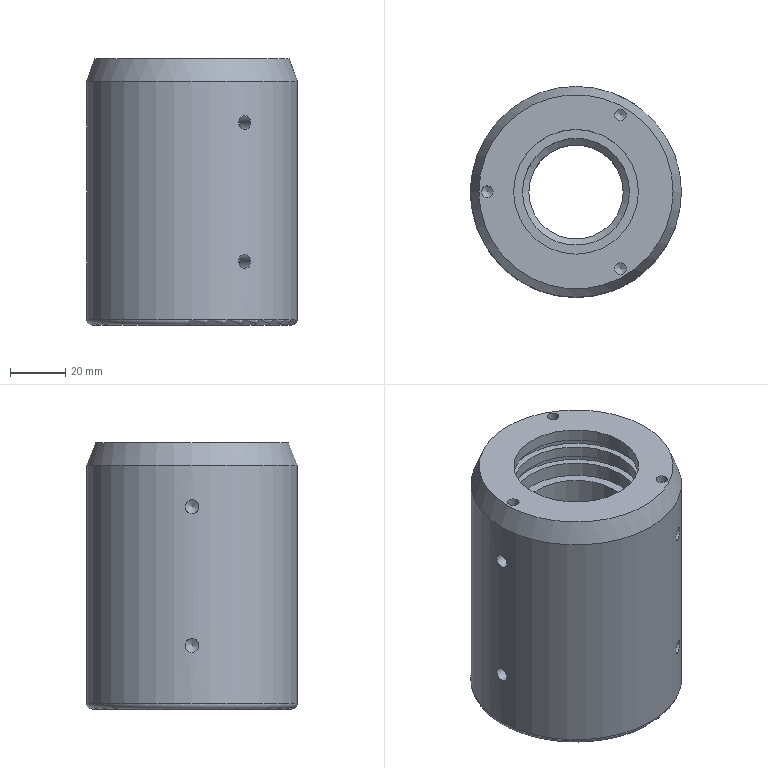Component | NX | CH3404_8-2 | 1 solid | 43 faces | volume 318375 mm3 | cylinder 20 | cone 14 | plane 7 | torus 2 | commonest cylinder face diameters 5 x9 45 x3 4.2 x3 49.6 x2 76 x1 34 x1 38.6 x1